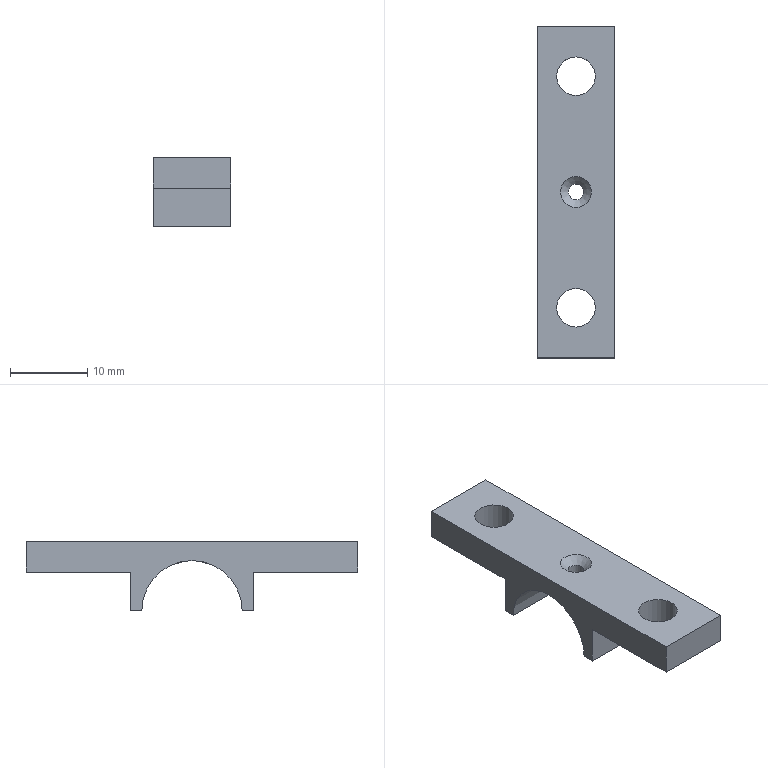Component | NX | 12B__27_3 | 1 solid | 16 faces | volume 1687 mm3 | plane 11 | cylinder 4 | cone 1 | commonest cylinder face diameters 5 x2 13 x1 2 x1